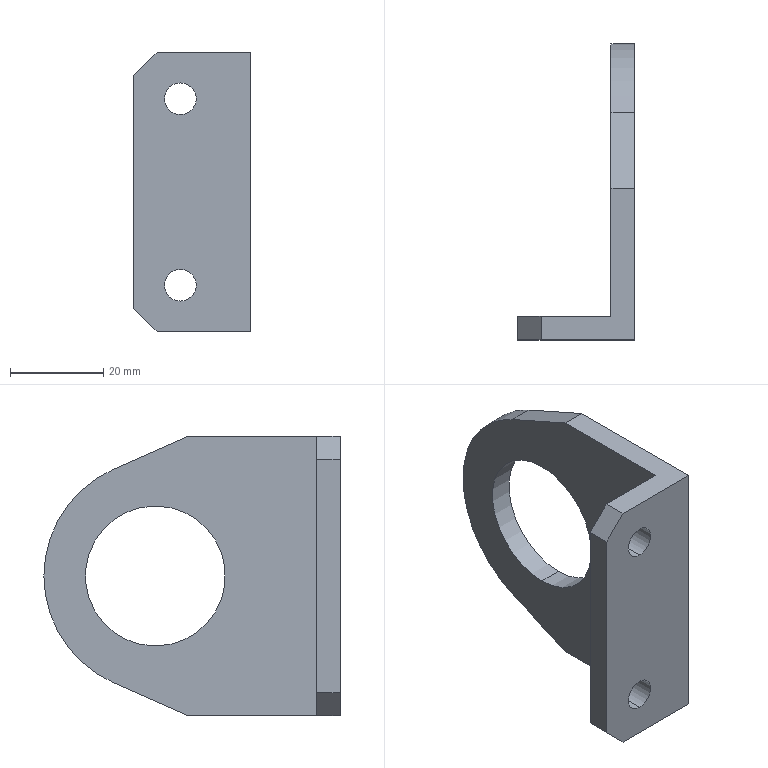Component | SolidWorks | FlipMechanismB-09-1 | 1 solid | 18 faces | box 25 x 63.5 x 60 mm | volume 18438 mm3 | plane 11 | cylinder 7 | commonest cylinder face diameters 6.8 x4 30 x2 50 x1
STEP:
#1=CARTESIAN_POINT('',(-0.5906,-1.559,-0.6535));
#2=VERTEX_POINT('',#1);
#3=CARTESIAN_POINT('',(-0.5906,-1.559,-0.9213));
#4=VERTEX_POINT('',#3);
#5=CARTESIAN_POINT('',(-0.5906,-1.559,-0.7874));
#6=DIRECTION('',(0.,1.,-0.));
#7=DIRECTION('',(0.,0.,-1.));
#8=AXIS2_PLACEMENT_3D('',#5,#6,#7);
#9=CIRCLE('',#8,0.1339);
#10=EDGE_CURVE('',#2,#4,#9,.T.);
#11=ORIENTED_EDGE('',*,*,#10,.F.);
#12=CARTESIAN_POINT('',(-0.5906,-1.362,-0.6535));
#13=VERTEX_POINT('',#12);
#14=CARTESIAN_POINT('',(-0.5906,-2.071,-0.6535));
#15=DIRECTION('',(0.,1.,0.));
#16=VECTOR('',#15,39.37);
#17=LINE('',#14,#16);
#18=EDGE_CURVE('',#2,#13,#17,.T.);
#19=ORIENTED_EDGE('',*,*,#18,.T.);
#20=CARTESIAN_POINT('',(-0.5906,-1.362,-0.9213));
#21=VERTEX_POINT('',#20);
#22=CARTESIAN_POINT('',(-0.5906,-1.362,-0.7874));
#23=DIRECTION('',(0.,1.,0.));
#24=DIRECTION('',(0.,0.,-1.));
#25=AXIS2_PLACEMENT_3D('',#22,#23,#24);
#26=CIRCLE('',#25,0.1339);
#27=EDGE_CURVE('',#13,#21,#26,.T.);
#28=ORIENTED_EDGE('',*,*,#27,.T.);
#29=CARTESIAN_POINT('',(-0.5906,-2.071,-0.9213));
#30=DIRECTION('',(0.,1.,0.));
#31=VECTOR('',#30,39.37);
#32=LINE('',#29,#31);
#33=EDGE_CURVE('',#4,#21,#32,.T.);
#34=ORIENTED_EDGE('',*,*,#33,.F.);
#35=EDGE_LOOP('',(#11,#19,#28,#34));
#36=FACE_OUTER_BOUND('',#35,.T.);
#37=CARTESIAN_POINT('',(-0.5906,-2.071,-0.7874));
#38=DIRECTION('',(0.,1.,0.));
#39=DIRECTION('',(0.,0.,-1.));
#40=AXIS2_PLACEMENT_3D('',#37,#38,#39);
#41=CYLINDRICAL_SURFACE('',#40,0.1339);
#42=ADVANCED_FACE('',(#36),#41,.F.);
#43=CARTESIAN_POINT('',(-0.5906,-1.559,0.9213));
#44=VERTEX_POINT('',#43);
#45=CARTESIAN_POINT('',(-0.5906,-1.559,0.6535));
#46=VERTEX_POINT('',#45);
#47=CARTESIAN_POINT('',(-0.5906,-1.559,0.7874));
#48=DIRECTION('',(0.,1.,-0.));
#49=DIRECTION('',(0.,0.,-1.));
#50=AXIS2_PLACEMENT_3D('',#47,#48,#49);
#51=CIRCLE('',#50,0.1339);
#52=EDGE_CURVE('',#44,#46,#51,.T.);
#53=ORIENTED_EDGE('',*,*,#52,.F.);
#54=CARTESIAN_POINT('',(-0.5906,-1.362,0.9213));
#55=VERTEX_POINT('',#54);
#56=CARTESIAN_POINT('',(-0.5906,-2.071,0.9213));
#57=DIRECTION('',(0.,1.,0.));
#58=VECTOR('',#57,39.37);
#59=LINE('',#56,#58);
#60=EDGE_CURVE('',#44,#55,#59,.T.);
#61=ORIENTED_EDGE('',*,*,#60,.T.);
#62=CARTESIAN_POINT('',(-0.5906,-1.362,0.6535));
#63=VERTEX_POINT('',#62);
#64=CARTESIAN_POINT('',(-0.5906,-1.362,0.7874));
#65=DIRECTION('',(0.,1.,0.));
#66=DIRECTION('',(0.,0.,-1.));
#67=AXIS2_PLACEMENT_3D('',#64,#65,#66);
#68=CIRCLE('',#67,0.1339);
#69=EDGE_CURVE('',#55,#63,#68,.T.);
#70=ORIENTED_EDGE('',*,*,#69,.T.);
#71=CARTESIAN_POINT('',(-0.5906,-2.071,0.6535));
#72=DIRECTION('',(0.,1.,0.));
#73=VECTOR('',#72,39.37);
#74=LINE('',#71,#73);
#75=EDGE_CURVE('',#46,#63,#74,.T.);
#76=ORIENTED_EDGE('',*,*,#75,.F.);
#77=EDGE_LOOP('',(#53,#61,#70,#76));
#78=FACE_OUTER_BOUND('',#77,.T.);
#79=CARTESIAN_POINT('',(-0.5906,-2.071,0.7874));
#80=DIRECTION('',(0.,1.,0.));
#81=DIRECTION('',(0.,0.,-1.));
#82=AXIS2_PLACEMENT_3D('',#79,#80,#81);
#83=CYLINDRICAL_SURFACE('',#82,0.1339);
#84=ADVANCED_FACE('',(#78),#83,.F.);
#85=CARTESIAN_POINT('',(0.,-0.,-0.5906));
#86=VERTEX_POINT('',#85);
#87=CARTESIAN_POINT('',(0.,-0.,0.5906));
#88=VERTEX_POINT('',#87);
#89=CARTESIAN_POINT('',(0.,-0.,-0.));
#90=DIRECTION('',(-1.,0.,0.));
#91=DIRECTION('',(0.,0.,1.));
#92=AXIS2_PLACEMENT_3D('',#89,#90,#91);
#93=CIRCLE('',#92,0.5906);
#94=EDGE_CURVE('',#86,#88,#93,.T.);
#95=ORIENTED_EDGE('',*,*,#94,.F.);
#96=CARTESIAN_POINT('',(-0.1969,-0.,-0.5906));
#97=VERTEX_POINT('',#96);
#98=CARTESIAN_POINT('',(0.,-0.,-0.5906));
#99=DIRECTION('',(-1.,0.,0.));
#100=VECTOR('',#99,39.37);
#101=LINE('',#98,#100);
#102=EDGE_CURVE('',#86,#97,#101,.T.);
#103=ORIENTED_EDGE('',*,*,#102,.T.);
#104=CARTESIAN_POINT('',(-0.1969,-0.,0.5906));
#105=VERTEX_POINT('',#104);
#106=CARTESIAN_POINT('',(-0.1969,-0.,-0.));
#107=DIRECTION('',(-1.,0.,0.));
#108=DIRECTION('',(0.,0.,1.));
#109=AXIS2_PLACEMENT_3D('',#106,#107,#108);
#110=CIRCLE('',#109,0.5906);
#111=EDGE_CURVE('',#97,#105,#110,.T.);
#112=ORIENTED_EDGE('',*,*,#111,.T.);
#113=CARTESIAN_POINT('',(0.,-0.,0.5906));
#114=DIRECTION('',(-1.,0.,0.));
#115=VECTOR('',#114,39.37);
#116=LINE('',#113,#115);
#117=EDGE_CURVE('',#88,#105,#116,.T.);
#118=ORIENTED_EDGE('',*,*,#117,.F.);
#119=EDGE_LOOP('',(#95,#103,#112,#118));
#120=FACE_OUTER_BOUND('',#119,.T.);
#121=CARTESIAN_POINT('',(0.,-0.,-0.));
#122=DIRECTION('',(-1.,0.,0.));
#123=DIRECTION('',(0.,0.,1.));
#124=AXIS2_PLACEMENT_3D('',#121,#122,#123);
#125=CYLINDRICAL_SURFACE('',#124,0.5906);
#126=ADVANCED_FACE('',(#120),#125,.F.);
#127=CARTESIAN_POINT('',(-0.1969,0.3553,-0.8999));
#128=VERTEX_POINT('',#127);
#129=CARTESIAN_POINT('',(-0.1969,-0.2795,-1.181));
#130=VERTEX_POINT('',#129);
#131=CARTESIAN_POINT('',(-0.1969,0.3553,-0.8999));
#132=DIRECTION('',(-0.,-0.9143,-0.405));
#133=VECTOR('',#132,39.37);
#134=LINE('',#131,#133);
#135=EDGE_CURVE('',#128,#130,#134,.T.);
#136=ORIENTED_EDGE('',*,*,#135,.F.);
#137=CARTESIAN_POINT('',(-0.,0.3553,-0.8999));
#138=VERTEX_POINT('',#137);
#139=CARTESIAN_POINT('',(-0.,0.3553,-0.8999));
#140=DIRECTION('',(-1.,0.,0.));
#141=VECTOR('',#140,39.37);
#142=LINE('',#139,#141);
#143=EDGE_CURVE('',#138,#128,#142,.T.);
#144=ORIENTED_EDGE('',*,*,#143,.F.);
#145=CARTESIAN_POINT('',(-0.,-0.2795,-1.181));
#146=VERTEX_POINT('',#145);
#147=CARTESIAN_POINT('',(-0.,0.3553,-0.8999));
#148=DIRECTION('',(-0.,-0.9143,-0.405));
#149=VECTOR('',#148,39.37);
#150=LINE('',#147,#149);
#151=EDGE_CURVE('',#138,#146,#150,.T.);
#152=ORIENTED_EDGE('',*,*,#151,.T.);
#153=CARTESIAN_POINT('',(-0.,-0.2795,-1.181));
#154=DIRECTION('',(-1.,0.,0.));
#155=VECTOR('',#154,39.37);
#156=LINE('',#153,#155);
#157=EDGE_CURVE('',#146,#130,#156,.T.);
#158=ORIENTED_EDGE('',*,*,#157,.T.);
#159=EDGE_LOOP('',(#136,#144,#152,#158));
#160=FACE_OUTER_BOUND('',#159,.T.);
#161=CARTESIAN_POINT('',(-0.,0.3553,-0.8999));
#162=DIRECTION('',(-0.,0.405,-0.9143));
#163=DIRECTION('',(-0.,-0.9143,-0.405));
#164=AXIS2_PLACEMENT_3D('',#161,#162,#163);
#165=PLANE('',#164);
#166=ADVANCED_FACE('',(#160),#165,.T.);
#167=CARTESIAN_POINT('',(-0.1969,0.3553,0.8999));
#168=VERTEX_POINT('',#167);
#169=CARTESIAN_POINT('',(-0.1969,-0.04331,0.));
#170=DIRECTION('',(-1.,0.,0.));
#171=DIRECTION('',(0.,0.,1.));
#172=AXIS2_PLACEMENT_3D('',#169,#170,#171);
#173=CIRCLE('',#172,0.9843);
#174=EDGE_CURVE('',#168,#128,#173,.T.);
#175=ORIENTED_EDGE('',*,*,#174,.F.);
#176=CARTESIAN_POINT('',(-0.,0.3553,0.8999));
#177=VERTEX_POINT('',#176);
#178=CARTESIAN_POINT('',(-0.,0.3553,0.8999));
#179=DIRECTION('',(-1.,0.,0.));
#180=VECTOR('',#179,39.37);
#181=LINE('',#178,#180);
#182=EDGE_CURVE('',#177,#168,#181,.T.);
#183=ORIENTED_EDGE('',*,*,#182,.F.);
#184=CARTESIAN_POINT('',(-0.,-0.04331,0.));
#185=DIRECTION('',(-1.,0.,0.));
#186=DIRECTION('',(0.,0.,1.));
#187=AXIS2_PLACEMENT_3D('',#184,#185,#186);
#188=CIRCLE('',#187,0.9843);
#189=EDGE_CURVE('',#177,#138,#188,.T.);
#190=ORIENTED_EDGE('',*,*,#189,.T.);
#191=ORIENTED_EDGE('',*,*,#143,.T.);
#192=EDGE_LOOP('',(#175,#183,#190,#191));
#193=FACE_OUTER_BOUND('',#192,.T.);
#194=CARTESIAN_POINT('',(-0.,-0.04331,0.));
#195=DIRECTION('',(-1.,0.,0.));
#196=DIRECTION('',(0.,0.,1.));
#197=AXIS2_PLACEMENT_3D('',#194,#195,#196);
#198=CYLINDRICAL_SURFACE('',#197,0.9843);
#199=ADVANCED_FACE('',(#193),#198,.T.);
#200=CARTESIAN_POINT('',(-0.1969,-0.2795,1.181));
#201=VERTEX_POINT('',#200);
#202=CARTESIAN_POINT('',(-0.1969,0.3553,0.8999));
#203=DIRECTION('',(0.,0.9143,-0.405));
#204=VECTOR('',#203,39.37);
#205=LINE('',#202,#204);
#206=EDGE_CURVE('',#201,#168,#205,.T.);
#207=ORIENTED_EDGE('',*,*,#206,.F.);
#208=CARTESIAN_POINT('',(-0.,-0.2795,1.181));
#209=VERTEX_POINT('',#208);
#210=CARTESIAN_POINT('',(-0.,-0.2795,1.181));
#211=DIRECTION('',(-1.,0.,0.));
#212=VECTOR('',#211,39.37);
#213=LINE('',#210,#212);
#214=EDGE_CURVE('',#209,#201,#213,.T.);
#215=ORIENTED_EDGE('',*,*,#214,.F.);
#216=CARTESIAN_POINT('',(-0.,0.3553,0.8999));
#217=DIRECTION('',(0.,0.9143,-0.405));
#218=VECTOR('',#217,39.37);
#219=LINE('',#216,#218);
#220=EDGE_CURVE('',#209,#177,#219,.T.);
#221=ORIENTED_EDGE('',*,*,#220,.T.);
#222=ORIENTED_EDGE('',*,*,#182,.T.);
#223=EDGE_LOOP('',(#207,#215,#221,#222));
#224=FACE_OUTER_BOUND('',#223,.T.);
#225=CARTESIAN_POINT('',(-0.,0.3553,0.8999));
#226=DIRECTION('',(0.,0.405,0.9143));
#227=DIRECTION('',(0.,0.9143,-0.405));
#228=AXIS2_PLACEMENT_3D('',#225,#226,#227);
#229=PLANE('',#228);
#230=ADVANCED_FACE('',(#224),#229,.T.);
#231=CARTESIAN_POINT('',(0.,-0.,-0.));
#232=DIRECTION('',(-1.,0.,0.));
#233=DIRECTION('',(0.,0.,1.));
#234=AXIS2_PLACEMENT_3D('',#231,#232,#233);
#235=CIRCLE('',#234,0.5906);
#236=EDGE_CURVE('',#88,#86,#235,.T.);
#237=ORIENTED_EDGE('',*,*,#236,.T.);
#238=ORIENTED_EDGE('',*,*,#94,.T.);
#239=EDGE_LOOP('',(#237,#238));
#240=FACE_BOUND('',#239,.T.);
#241=ORIENTED_EDGE('',*,*,#220,.F.);
#242=CARTESIAN_POINT('',(-0.,-1.559,1.181));
#243=VERTEX_POINT('',#242);
#244=CARTESIAN_POINT('',(-0.,-1.559,1.181));
#245=DIRECTION('',(0.,1.,-0.));
#246=VECTOR('',#245,39.37);
#247=LINE('',#244,#246);
#248=EDGE_CURVE('',#243,#209,#247,.T.);
#249=ORIENTED_EDGE('',*,*,#248,.F.);
#250=CARTESIAN_POINT('',(0.,-1.559,-1.181));
#251=VERTEX_POINT('',#250);
#252=CARTESIAN_POINT('',(0.,-1.559,-1.181));
#253=DIRECTION('',(-0.,0.,1.));
#254=VECTOR('',#253,39.37);
#255=LINE('',#252,#254);
#256=EDGE_CURVE('',#251,#243,#255,.T.);
#257=ORIENTED_EDGE('',*,*,#256,.F.);
#258=CARTESIAN_POINT('',(0.,-1.559,-1.181));
#259=DIRECTION('',(0.,1.,-0.));
#260=VECTOR('',#259,39.37);
#261=LINE('',#258,#260);
#262=EDGE_CURVE('',#251,#146,#261,.T.);
#263=ORIENTED_EDGE('',*,*,#262,.T.);
#264=ORIENTED_EDGE('',*,*,#151,.F.);
#265=ORIENTED_EDGE('',*,*,#189,.F.);
#266=EDGE_LOOP('',(#241,#249,#257,#263,#264,#265));
#267=FACE_OUTER_BOUND('',#266,.T.);
#268=CARTESIAN_POINT('',(-0.,-0.04331,0.));
#269=DIRECTION('',(-1.,0.,0.));
#270=DIRECTION('',(0.,0.,1.));
#271=AXIS2_PLACEMENT_3D('',#268,#269,#270);
#272=PLANE('',#271);
#273=ADVANCED_FACE('',(#240,#267),#272,.F.);
#274=CARTESIAN_POINT('',(-0.1969,-0.,-0.));
#275=DIRECTION('',(-1.,0.,0.));
#276=DIRECTION('',(0.,0.,1.));
#277=AXIS2_PLACEMENT_3D('',#274,#275,#276);
#278=CIRCLE('',#277,0.5906);
#279=EDGE_CURVE('',#105,#97,#278,.T.);
#280=ORIENTED_EDGE('',*,*,#279,.F.);
#281=ORIENTED_EDGE('',*,*,#111,.F.);
#282=EDGE_LOOP('',(#280,#281));
#283=FACE_BOUND('',#282,.T.);
#284=CARTESIAN_POINT('',(-0.1969,-1.362,1.181));
#285=VERTEX_POINT('',#284);
#286=CARTESIAN_POINT('',(-0.1969,-1.362,-1.181));
#287=VERTEX_POINT('',#286);
#288=CARTESIAN_POINT('',(-0.1969,-1.362,-0.));
#289=DIRECTION('',(-0.,0.,-1.));
#290=VECTOR('',#289,39.37);
#291=LINE('',#288,#290);
#292=EDGE_CURVE('',#285,#287,#291,.T.);
#293=ORIENTED_EDGE('',*,*,#292,.F.);
#294=CARTESIAN_POINT('',(-0.1969,-1.559,1.181));
#295=DIRECTION('',(0.,1.,-0.));
#296=VECTOR('',#295,39.37);
#297=LINE('',#294,#296);
#298=EDGE_CURVE('',#285,#201,#297,.T.);
#299=ORIENTED_EDGE('',*,*,#298,.T.);
#300=ORIENTED_EDGE('',*,*,#206,.T.);
#301=ORIENTED_EDGE('',*,*,#174,.T.);
#302=ORIENTED_EDGE('',*,*,#135,.T.);
#303=CARTESIAN_POINT('',(-0.1969,-1.559,-1.181));
#304=DIRECTION('',(0.,1.,-0.));
#305=VECTOR('',#304,39.37);
#306=LINE('',#303,#305);
#307=EDGE_CURVE('',#287,#130,#306,.T.);
#308=ORIENTED_EDGE('',*,*,#307,.F.);
#309=EDGE_LOOP('',(#293,#299,#300,#301,#302,#308));
#310=FACE_OUTER_BOUND('',#309,.T.);
#311=CARTESIAN_POINT('',(-0.1969,-0.04331,0.));
#312=DIRECTION('',(-1.,0.,0.));
#313=DIRECTION('',(0.,0.,1.));
#314=AXIS2_PLACEMENT_3D('',#311,#312,#313);
#315=PLANE('',#314);
#316=ADVANCED_FACE('',(#283,#310),#315,.T.);
#317=CARTESIAN_POINT('',(-0.7874,-1.559,-1.181));
#318=VERTEX_POINT('',#317);
#319=CARTESIAN_POINT('',(-0.1969,-1.559,-1.181));
#320=DIRECTION('',(1.,0.,0.));
#321=VECTOR('',#320,39.37);
#322=LINE('',#319,#321);
#323=EDGE_CURVE('',#318,#251,#322,.T.);
#324=ORIENTED_EDGE('',*,*,#323,.F.);
#325=CARTESIAN_POINT('',(-0.7874,-1.362,-1.181));
#326=VERTEX_POINT('',#325);
#327=CARTESIAN_POINT('',(-0.7874,-1.362,-1.181));
#328=DIRECTION('',(0.,1.,-0.));
#329=VECTOR('',#328,39.37);
#330=LINE('',#327,#329);
#331=EDGE_CURVE('',#318,#326,#330,.T.);
#332=ORIENTED_EDGE('',*,*,#331,.T.);
#333=CARTESIAN_POINT('',(-0.9843,-1.362,-1.181));
#334=DIRECTION('',(1.,0.,0.));
#335=VECTOR('',#334,39.37);
#336=LINE('',#333,#335);
#337=EDGE_CURVE('',#326,#287,#336,.T.);
#338=ORIENTED_EDGE('',*,*,#337,.T.);
#339=ORIENTED_EDGE('',*,*,#307,.T.);
#340=ORIENTED_EDGE('',*,*,#157,.F.);
#341=ORIENTED_EDGE('',*,*,#262,.F.);
#342=EDGE_LOOP('',(#324,#332,#338,#339,#340,#341));
#343=FACE_OUTER_BOUND('',#342,.T.);
#344=CARTESIAN_POINT('',(-0.1969,-1.559,-1.181));
#345=DIRECTION('',(0.,0.,1.));
#346=DIRECTION('',(0.,1.,-0.));
#347=AXIS2_PLACEMENT_3D('',#344,#345,#346);
#348=PLANE('',#347);
#349=ADVANCED_FACE('',(#343),#348,.F.);
#350=CARTESIAN_POINT('',(-0.7874,-1.362,1.181));
#351=VERTEX_POINT('',#350);
#352=CARTESIAN_POINT('',(-0.9843,-1.362,1.181));
#353=DIRECTION('',(1.,0.,0.));
#354=VECTOR('',#353,39.37);
#355=LINE('',#352,#354);
#356=EDGE_CURVE('',#351,#285,#355,.T.);
#357=ORIENTED_EDGE('',*,*,#356,.F.);
#358=CARTESIAN_POINT('',(-0.7874,-1.559,1.181));
#359=VERTEX_POINT('',#358);
#360=CARTESIAN_POINT('',(-0.7874,-1.559,1.181));
#361=DIRECTION('',(-0.,-1.,0.));
#362=VECTOR('',#361,39.37);
#363=LINE('',#360,#362);
#364=EDGE_CURVE('',#351,#359,#363,.T.);
#365=ORIENTED_EDGE('',*,*,#364,.T.);
#366=CARTESIAN_POINT('',(-0.1969,-1.559,1.181));
#367=DIRECTION('',(-1.,0.,0.));
#368=VECTOR('',#367,39.37);
#369=LINE('',#366,#368);
#370=EDGE_CURVE('',#243,#359,#369,.T.);
#371=ORIENTED_EDGE('',*,*,#370,.F.);
#372=ORIENTED_EDGE('',*,*,#248,.T.);
#373=ORIENTED_EDGE('',*,*,#214,.T.);
#374=ORIENTED_EDGE('',*,*,#298,.F.);
#375=EDGE_LOOP('',(#357,#365,#371,#372,#373,#374));
#376=FACE_OUTER_BOUND('',#375,.T.);
#377=CARTESIAN_POINT('',(-0.1969,-1.559,1.181));
#378=DIRECTION('',(-0.,-0.,-1.));
#379=DIRECTION('',(-0.,-1.,0.));
#380=AXIS2_PLACEMENT_3D('',#377,#378,#379);
#381=PLANE('',#380);
#382=ADVANCED_FACE('',(#376),#381,.F.);
#383=CARTESIAN_POINT('',(-0.5906,-1.559,-0.7874));
#384=DIRECTION('',(0.,1.,-0.));
#385=DIRECTION('',(0.,0.,-1.));
#386=AXIS2_PLACEMENT_3D('',#383,#384,#385);
#387=CIRCLE('',#386,0.1339);
#388=EDGE_CURVE('',#4,#2,#387,.T.);
#389=ORIENTED_EDGE('',*,*,#388,.T.);
#390=ORIENTED_EDGE('',*,*,#10,.T.);
#391=EDGE_LOOP('',(#389,#390));
#392=FACE_BOUND('',#391,.T.);
#393=CARTESIAN_POINT('',(-0.5906,-1.559,0.7874));
#394=DIRECTION('',(0.,1.,-0.));
#395=DIRECTION('',(0.,0.,-1.));
#396=AXIS2_PLACEMENT_3D('',#393,#394,#395);
#397=CIRCLE('',#396,0.1339);
#398=EDGE_CURVE('',#46,#44,#397,.T.);
#399=ORIENTED_EDGE('',*,*,#398,.T.);
#400=ORIENTED_EDGE('',*,*,#52,.T.);
#401=EDGE_LOOP('',(#399,#400));
#402=FACE_BOUND('',#401,.T.);
#403=CARTESIAN_POINT('',(-0.9843,-1.559,0.9843));
#404=VERTEX_POINT('',#403);
#405=CARTESIAN_POINT('',(-0.9843,-1.559,-0.9843));
#406=VERTEX_POINT('',#405);
#407=CARTESIAN_POINT('',(-0.9843,-1.559,-1.181));
#408=DIRECTION('',(-0.,-0.,-1.));
#409=VECTOR('',#408,39.37);
#410=LINE('',#407,#409);
#411=EDGE_CURVE('',#404,#406,#410,.T.);
#412=ORIENTED_EDGE('',*,*,#411,.T.);
#413=CARTESIAN_POINT('',(-0.7874,-1.559,-1.181));
#414=DIRECTION('',(0.7071,-0.,-0.7071));
#415=VECTOR('',#414,39.37);
#416=LINE('',#413,#415);
#417=EDGE_CURVE('',#406,#318,#416,.T.);
#418=ORIENTED_EDGE('',*,*,#417,.T.);
#419=ORIENTED_EDGE('',*,*,#323,.T.);
#420=ORIENTED_EDGE('',*,*,#256,.T.);
#421=ORIENTED_EDGE('',*,*,#370,.T.);
#422=CARTESIAN_POINT('',(-0.7874,-1.559,1.181));
#423=DIRECTION('',(-0.7071,-0.,-0.7071));
#424=VECTOR('',#423,39.37);
#425=LINE('',#422,#424);
#426=EDGE_CURVE('',#359,#404,#425,.T.);
#427=ORIENTED_EDGE('',*,*,#426,.T.);
#428=EDGE_LOOP('',(#412,#418,#419,#420,#421,#427));
#429=FACE_OUTER_BOUND('',#428,.T.);
#430=CARTESIAN_POINT('',(-0.1969,-1.559,0.));
#431=DIRECTION('',(0.,1.,-0.));
#432=DIRECTION('',(-0.,-0.,-1.));
#433=AXIS2_PLACEMENT_3D('',#430,#431,#432);
#434=PLANE('',#433);
#435=ADVANCED_FACE('',(#392,#402,#429),#434,.F.);
#436=CARTESIAN_POINT('',(-0.5906,-1.362,-0.7874));
#437=DIRECTION('',(0.,1.,0.));
#438=DIRECTION('',(0.,0.,-1.));
#439=AXIS2_PLACEMENT_3D('',#436,#437,#438);
#440=CIRCLE('',#439,0.1339);
#441=EDGE_CURVE('',#21,#13,#440,.T.);
#442=ORIENTED_EDGE('',*,*,#441,.F.);
#443=ORIENTED_EDGE('',*,*,#27,.F.);
#444=EDGE_LOOP('',(#442,#443));
#445=FACE_BOUND('',#444,.T.);
#446=CARTESIAN_POINT('',(-0.5906,-1.362,0.7874));
#447=DIRECTION('',(0.,1.,0.));
#448=DIRECTION('',(0.,0.,-1.));
#449=AXIS2_PLACEMENT_3D('',#446,#447,#448);
#450=CIRCLE('',#449,0.1339);
#451=EDGE_CURVE('',#63,#55,#450,.T.);
#452=ORIENTED_EDGE('',*,*,#451,.F.);
#453=ORIENTED_EDGE('',*,*,#69,.F.);
#454=EDGE_LOOP('',(#452,#453));
#455=FACE_BOUND('',#454,.T.);
#456=ORIENTED_EDGE('',*,*,#337,.F.);
#457=CARTESIAN_POINT('',(-0.9843,-1.362,-0.9843));
#458=VERTEX_POINT('',#457);
#459=CARTESIAN_POINT('',(-0.8858,-1.362,-1.083));
#460=DIRECTION('',(-0.7071,-0.,0.7071));
#461=VECTOR('',#460,39.37);
#462=LINE('',#459,#461);
#463=EDGE_CURVE('',#326,#458,#462,.T.);
#464=ORIENTED_EDGE('',*,*,#463,.T.);
#465=CARTESIAN_POINT('',(-0.9843,-1.362,0.9843));
#466=VERTEX_POINT('',#465);
#467=CARTESIAN_POINT('',(-0.9843,-1.362,-1.181));
#468=DIRECTION('',(0.,-0.,1.));
#469=VECTOR('',#468,39.37);
#470=LINE('',#467,#469);
#471=EDGE_CURVE('',#458,#466,#470,.T.);
#472=ORIENTED_EDGE('',*,*,#471,.T.);
#473=CARTESIAN_POINT('',(-2.067,-1.362,-0.09843));
#474=DIRECTION('',(0.7071,-0.,0.7071));
#475=VECTOR('',#474,39.37);
#476=LINE('',#473,#475);
#477=EDGE_CURVE('',#466,#351,#476,.T.);
#478=ORIENTED_EDGE('',*,*,#477,.T.);
#479=ORIENTED_EDGE('',*,*,#356,.T.);
#480=ORIENTED_EDGE('',*,*,#292,.T.);
#481=EDGE_LOOP('',(#456,#464,#472,#478,#479,#480));
#482=FACE_OUTER_BOUND('',#481,.T.);
#483=CARTESIAN_POINT('',(-0.9843,-1.362,-1.181));
#484=DIRECTION('',(0.,1.,0.));
#485=DIRECTION('',(-0.,0.,-1.));
#486=AXIS2_PLACEMENT_3D('',#483,#484,#485);
#487=PLANE('',#486);
#488=ADVANCED_FACE('',(#445,#455,#482),#487,.T.);
#489=ORIENTED_EDGE('',*,*,#471,.F.);
#490=CARTESIAN_POINT('',(-0.9843,-1.559,-0.9843));
#491=DIRECTION('',(-0.,-1.,0.));
#492=VECTOR('',#491,39.37);
#493=LINE('',#490,#492);
#494=EDGE_CURVE('',#458,#406,#493,.T.);
#495=ORIENTED_EDGE('',*,*,#494,.T.);
#496=ORIENTED_EDGE('',*,*,#411,.F.);
#497=CARTESIAN_POINT('',(-0.9843,-1.362,0.9843));
#498=DIRECTION('',(0.,1.,-0.));
#499=VECTOR('',#498,39.37);
#500=LINE('',#497,#499);
#501=EDGE_CURVE('',#404,#466,#500,.T.);
#502=ORIENTED_EDGE('',*,*,#501,.T.);
#503=EDGE_LOOP('',(#489,#495,#496,#502));
#504=FACE_OUTER_BOUND('',#503,.T.);
#505=CARTESIAN_POINT('',(-0.9843,-0.04331,0.));
#506=DIRECTION('',(-1.,0.,0.));
#507=DIRECTION('',(0.,0.,1.));
#508=AXIS2_PLACEMENT_3D('',#505,#506,#507);
#509=PLANE('',#508);
#510=ADVANCED_FACE('',(#504),#509,.T.);
#511=ORIENTED_EDGE('',*,*,#102,.F.);
#512=ORIENTED_EDGE('',*,*,#236,.F.);
#513=ORIENTED_EDGE('',*,*,#117,.T.);
#514=ORIENTED_EDGE('',*,*,#279,.T.);
#515=EDGE_LOOP('',(#511,#512,#513,#514));
#516=FACE_OUTER_BOUND('',#515,.T.);
#517=CARTESIAN_POINT('',(0.,-0.,-0.));
#518=DIRECTION('',(-1.,0.,0.));
#519=DIRECTION('',(0.,0.,1.));
#520=AXIS2_PLACEMENT_3D('',#517,#518,#519);
#521=CYLINDRICAL_SURFACE('',#520,0.5906);
#522=ADVANCED_FACE('',(#516),#521,.F.);
#523=ORIENTED_EDGE('',*,*,#417,.F.);
#524=ORIENTED_EDGE('',*,*,#494,.F.);
#525=ORIENTED_EDGE('',*,*,#463,.F.);
#526=ORIENTED_EDGE('',*,*,#331,.F.);
#527=EDGE_LOOP('',(#523,#524,#525,#526));
#528=FACE_OUTER_BOUND('',#527,.T.);
#529=CARTESIAN_POINT('',(-0.7874,-1.559,-1.181));
#530=DIRECTION('',(-0.7071,-0.,-0.7071));
#531=DIRECTION('',(-0.,-1.,0.));
#532=AXIS2_PLACEMENT_3D('',#529,#530,#531);
#533=PLANE('',#532);
#534=ADVANCED_FACE('',(#528),#533,.T.);
#535=ORIENTED_EDGE('',*,*,#477,.F.);
#536=ORIENTED_EDGE('',*,*,#501,.F.);
#537=ORIENTED_EDGE('',*,*,#426,.F.);
#538=ORIENTED_EDGE('',*,*,#364,.F.);
#539=EDGE_LOOP('',(#535,#536,#537,#538));
#540=FACE_OUTER_BOUND('',#539,.T.);
#541=CARTESIAN_POINT('',(-0.7874,-1.559,1.181));
#542=DIRECTION('',(-0.7071,0.,0.7071));
#543=DIRECTION('',(0.,1.,-0.));
#544=AXIS2_PLACEMENT_3D('',#541,#542,#543);
#545=PLANE('',#544);
#546=ADVANCED_FACE('',(#540),#545,.T.);
#547=ORIENTED_EDGE('',*,*,#60,.F.);
#548=ORIENTED_EDGE('',*,*,#398,.F.);
#549=ORIENTED_EDGE('',*,*,#75,.T.);
#550=ORIENTED_EDGE('',*,*,#451,.T.);
#551=EDGE_LOOP('',(#547,#548,#549,#550));
#552=FACE_OUTER_BOUND('',#551,.T.);
#553=CARTESIAN_POINT('',(-0.5906,-2.071,0.7874));
#554=DIRECTION('',(0.,1.,0.));
#555=DIRECTION('',(0.,0.,-1.));
#556=AXIS2_PLACEMENT_3D('',#553,#554,#555);
#557=CYLINDRICAL_SURFACE('',#556,0.1339);
#558=ADVANCED_FACE('',(#552),#557,.F.);
#559=ORIENTED_EDGE('',*,*,#18,.F.);
#560=ORIENTED_EDGE('',*,*,#388,.F.);
#561=ORIENTED_EDGE('',*,*,#33,.T.);
#562=ORIENTED_EDGE('',*,*,#441,.T.);
#563=EDGE_LOOP('',(#559,#560,#561,#562));
#564=FACE_OUTER_BOUND('',#563,.T.);
#565=CARTESIAN_POINT('',(-0.5906,-2.071,-0.7874));
#566=DIRECTION('',(0.,1.,0.));
#567=DIRECTION('',(0.,0.,-1.));
#568=AXIS2_PLACEMENT_3D('',#565,#566,#567);
#569=CYLINDRICAL_SURFACE('',#568,0.1339);
#570=ADVANCED_FACE('',(#564),#569,.F.);
#571=CLOSED_SHELL('',(#42,#84,#126,#166,#199,#230,#273,#316,#349,#382,#435,#488,#510,#522,#534,#546,#558,#570));
#572=MANIFOLD_SOLID_BREP('',#571);
#573=CARTESIAN_POINT('',(0.,0.,0.));
#574=DIRECTION('',(0.,0.,1.));
#575=DIRECTION('',(1.,0.,0.));
#576=AXIS2_PLACEMENT_3D('',#573,#574,#575);
#577=(LENGTH_UNIT()NAMED_UNIT(*)SI_UNIT($,.METRE.));
#578=LENGTH_MEASURE_WITH_UNIT(LENGTH_MEASURE(0.0254),#577);
#579=DIMENSIONAL_EXPONENTS(1.,0.,0.,0.,0.,0.,0.);
#580=(CONVERSION_BASED_UNIT('',#578)LENGTH_UNIT()NAMED_UNIT(#579));
#581=UNCERTAINTY_MEASURE_WITH_UNIT(LENGTH_MEASURE(0.00001),#580,'','');
#582=(NAMED_UNIT(*)PLANE_ANGLE_UNIT()SI_UNIT($,.RADIAN.));
#583=(NAMED_UNIT(*)SI_UNIT($,.STERADIAN.)SOLID_ANGLE_UNIT());
#584=(GEOMETRIC_REPRESENTATION_CONTEXT(3)GLOBAL_UNCERTAINTY_ASSIGNED_CONTEXT((#581))GLOBAL_UNIT_ASSIGNED_CONTEXT((#580,#582,#583))REPRESENTATION_CONTEXT('',''));
#585=ADVANCED_BREP_SHAPE_REPRESENTATION('',(#572,#576),#584);
#586=COLOUR_RGB('',0.7922,0.8196,0.9333);
#587=FILL_AREA_STYLE_COLOUR('',#586);
#588=FILL_AREA_STYLE('',(#587));
#589=SURFACE_STYLE_FILL_AREA(#588);
#590=SURFACE_SIDE_STYLE('',(#589));
#591=SURFACE_STYLE_USAGE(.BOTH.,#590);
#592=PRESENTATION_STYLE_ASSIGNMENT((#591));
#593=STYLED_ITEM('',(#592),#572);
#594=(LENGTH_UNIT()NAMED_UNIT(*)SI_UNIT($,.METRE.));
#595=LENGTH_MEASURE_WITH_UNIT(LENGTH_MEASURE(0.0254),#594);
#596=DIMENSIONAL_EXPONENTS(1.,0.,0.,0.,0.,0.,0.);
#597=(CONVERSION_BASED_UNIT('',#595)LENGTH_UNIT()NAMED_UNIT(#596));
#598=UNCERTAINTY_MEASURE_WITH_UNIT(LENGTH_MEASURE(0.00001),#597,'','');
#599=(NAMED_UNIT(*)PLANE_ANGLE_UNIT()SI_UNIT($,.RADIAN.));
#600=(NAMED_UNIT(*)SI_UNIT($,.STERADIAN.)SOLID_ANGLE_UNIT());
#601=(GEOMETRIC_REPRESENTATION_CONTEXT(3)GLOBAL_UNCERTAINTY_ASSIGNED_CONTEXT((#598))GLOBAL_UNIT_ASSIGNED_CONTEXT((#597,#599,#600))REPRESENTATION_CONTEXT('',''));
#602=MECHANICAL_DESIGN_GEOMETRIC_PRESENTATION_REPRESENTATION('',(#593),#601);
#603=PRESENTATION_LAYER_ASSIGNMENT('','',(#593));